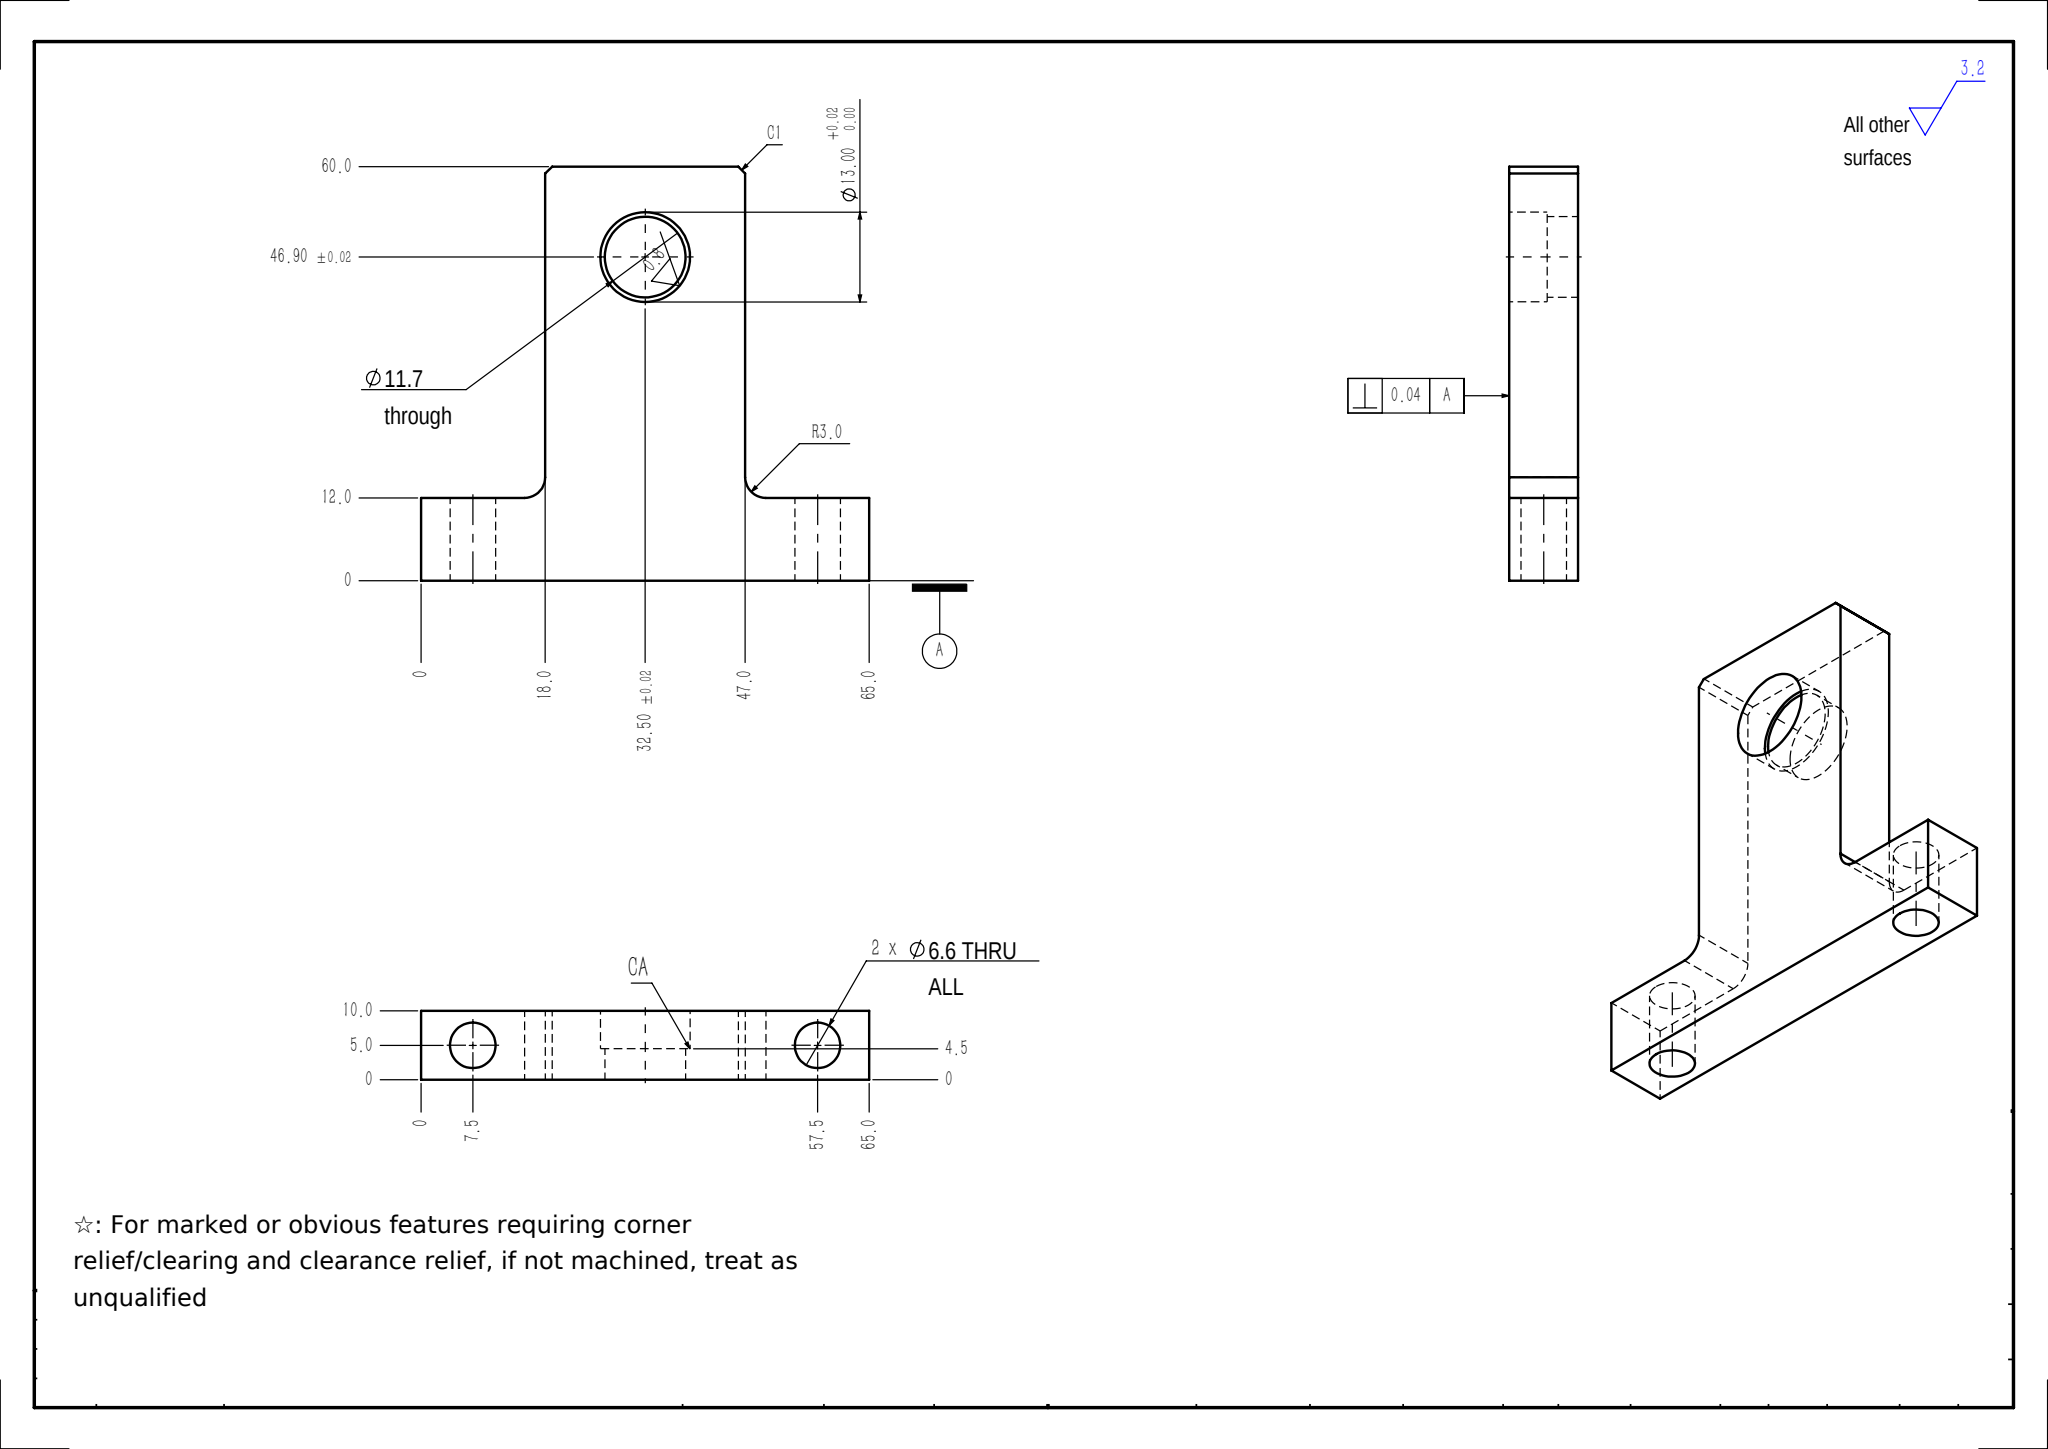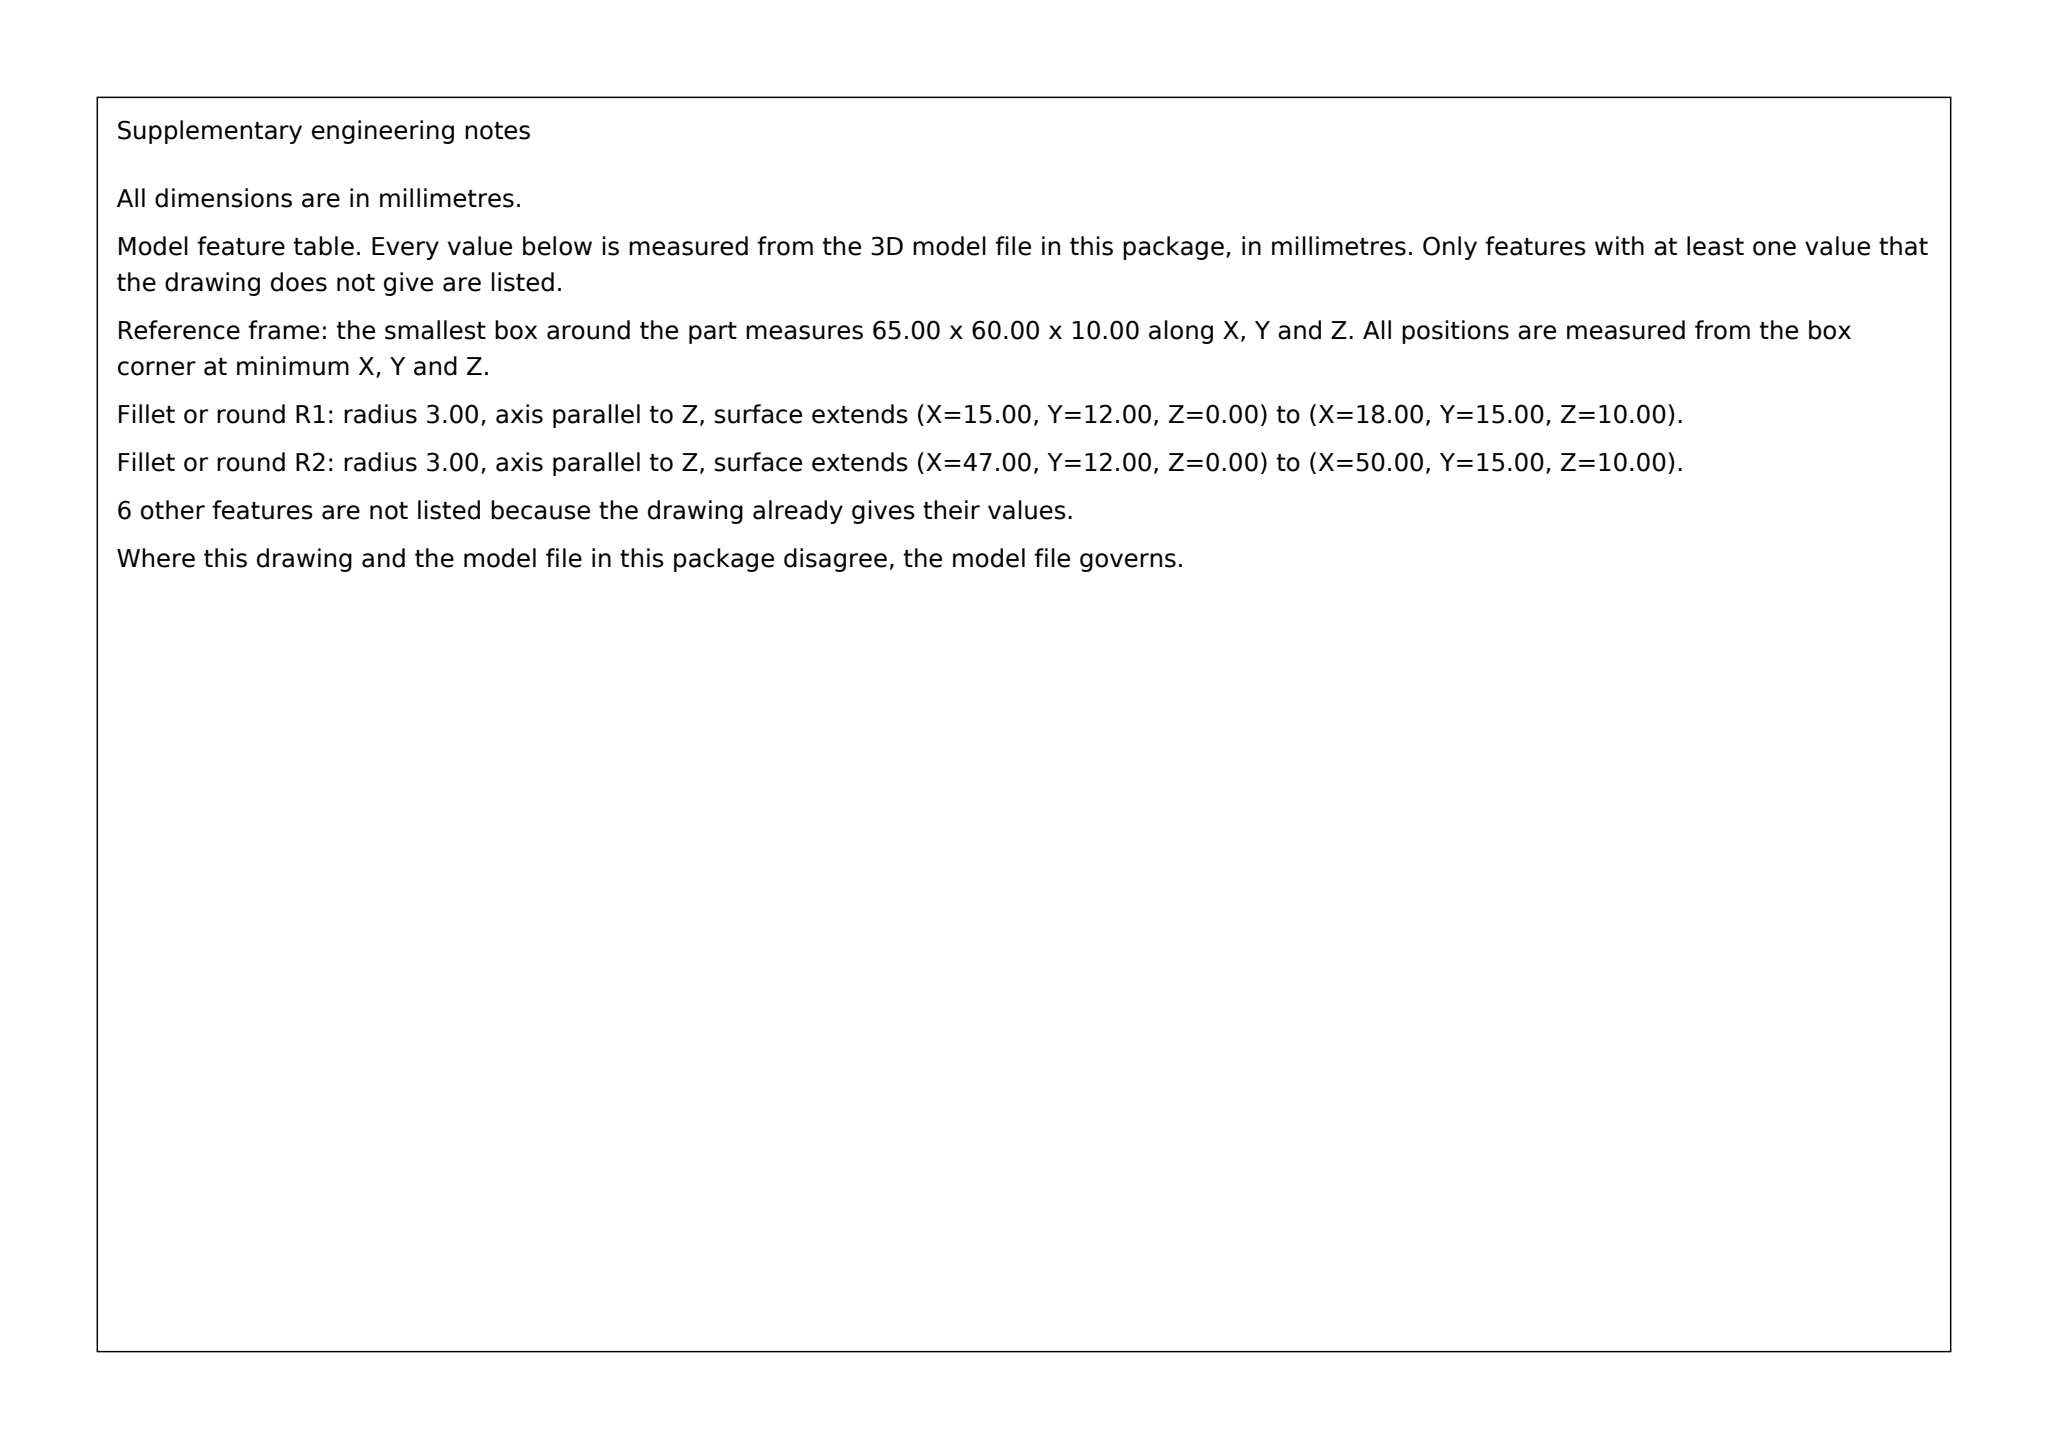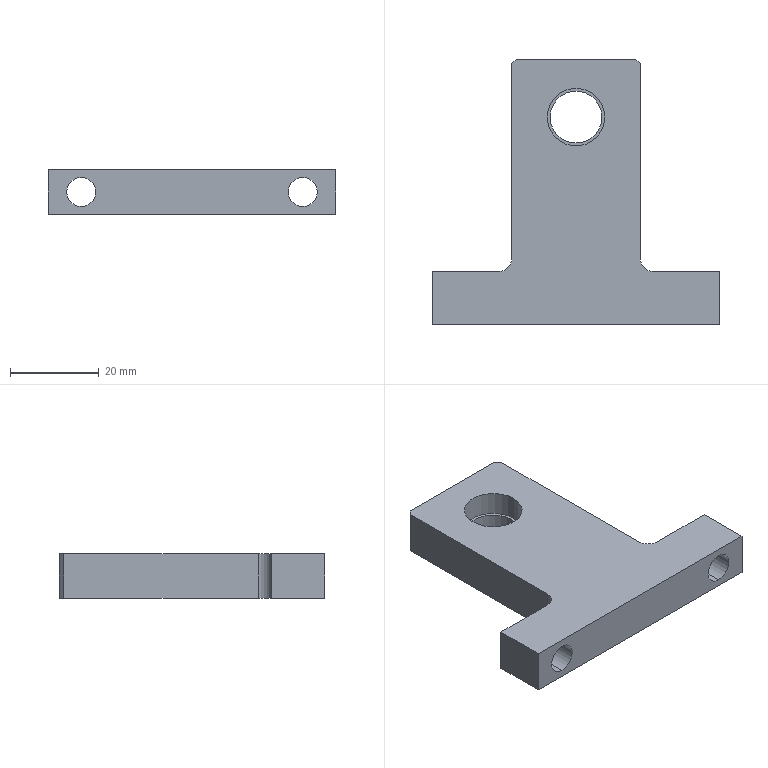Part | SolidWorks | mm | 1 solid | 23 faces | box 65 x 60 x 10 mm | volume 19714 mm3 | plane 13 | cylinder 10 | commonest cylinder face diameters 6.6 x4 11.7 x2 13 x2 6 x2
build123d program:
from build123d import *

# Parameters (mm, degrees)
BOSS_EXTRUDE1_DEPTH  = 5
FILLET1_R            = 3
SKETCH3_R            = 6.5
CUT_EXTRUDE1_DEPTH   = 46.346
SKETCH2_R            = 6.5
SKETCH2_R_2          = 5.85
BOSS_EXTRUDE2_DEPTH  = 4.5
M6_CLEARANCE_HOLE1_D = 6.6
CHAMFER1_SIZE        = 1


with BuildPart() as part:
    # Sketch1 → Boss-Extrude1 (new, symmetric)
    with BuildSketch(Plane.XY):
        Polygon((-14.5, 30), (-14.5, -18), (-32.5, -18), (-32.5, -30), (32.5, -30), (32.5, -18), (14.5, -18), (14.5, 30), align=None)
    extrude(amount=BOSS_EXTRUDE1_DEPTH, both=True)

    # Fillet1
    fillet1_edges = [part.edges().sort_by_distance(p)[0] for p in [
        (-14.5, -18, 0),
        (14.5, -18, 0),
    ]]
    fillet(fillet1_edges, radius=FILLET1_R)

    # Sketch3 → Cut-Extrude1 (cut, through all)
    with BuildSketch(Plane(origin=(0, 0, -5), x_dir=(-1, 0, 0), z_dir=(0, 0, -1))):
        with Locations((0, 16.9)):
            Circle(SKETCH3_R)
    extrude(amount=-CUT_EXTRUDE1_DEPTH, mode=Mode.SUBTRACT)

    # Sketch2 → Boss-Extrude2 (add)
    with BuildSketch(Plane(origin=(0, 0, -5), x_dir=(-1, 0, 0), z_dir=(0, 0, -1))):
        with Locations((0, 16.9)):
            Circle(SKETCH2_R)
        with Locations((0, 16.9)):
            Circle(SKETCH2_R_2, mode=Mode.SUBTRACT)
    extrude(amount=-BOSS_EXTRUDE2_DEPTH)

    # M6 Clearance Hole1 (through all)
    with Locations(Plane(origin=(0, -18, 0), x_dir=(1, 0, 0), z_dir=(0, 1, 0))):
        with Locations((-25, 0), (25, 0)):
            Hole(M6_CLEARANCE_HOLE1_D / 2)

    # Chamfer1
    chamfer1_edges = [part.edges().sort_by_distance(p)[0] for p in [
        (-14.5, 30, 0),
        (14.5, 30, 0),
    ]]
    chamfer(chamfer1_edges, length=CHAMFER1_SIZE)


solid = part.part
STEP:
#1=CARTESIAN_POINT('',(-25.,-30.,-3.3));
#2=VERTEX_POINT('',#1);
#3=CARTESIAN_POINT('',(-25.,-30.,3.3));
#4=VERTEX_POINT('',#3);
#5=CARTESIAN_POINT('',(-25.,-30.,0.));
#6=DIRECTION('',(0.,1.,0.));
#7=DIRECTION('',(0.,0.,1.));
#8=AXIS2_PLACEMENT_3D('',#5,#6,#7);
#9=CIRCLE('',#8,3.3);
#10=EDGE_CURVE('',#2,#4,#9,.T.);
#11=ORIENTED_EDGE('',*,*,#10,.F.);
#12=CARTESIAN_POINT('',(-25.,-18.,-3.3));
#13=VERTEX_POINT('',#12);
#14=CARTESIAN_POINT('',(-25.,-18.,-3.3));
#15=DIRECTION('',(0.,1.,0.));
#16=VECTOR('',#15,1000.);
#17=LINE('',#14,#16);
#18=EDGE_CURVE('',#2,#13,#17,.T.);
#19=ORIENTED_EDGE('',*,*,#18,.T.);
#20=CARTESIAN_POINT('',(-25.,-18.,3.3));
#21=VERTEX_POINT('',#20);
#22=CARTESIAN_POINT('',(-25.,-18.,0.));
#23=DIRECTION('',(0.,1.,0.));
#24=DIRECTION('',(0.,0.,1.));
#25=AXIS2_PLACEMENT_3D('',#22,#23,#24);
#26=CIRCLE('',#25,3.3);
#27=EDGE_CURVE('',#13,#21,#26,.T.);
#28=ORIENTED_EDGE('',*,*,#27,.T.);
#29=CARTESIAN_POINT('',(-25.,-18.,3.3));
#30=DIRECTION('',(0.,1.,0.));
#31=VECTOR('',#30,1000.);
#32=LINE('',#29,#31);
#33=EDGE_CURVE('',#4,#21,#32,.T.);
#34=ORIENTED_EDGE('',*,*,#33,.F.);
#35=EDGE_LOOP('',(#11,#19,#28,#34));
#36=FACE_OUTER_BOUND('',#35,.T.);
#37=CARTESIAN_POINT('',(-25.,-18.,0.));
#38=DIRECTION('',(0.,1.,0.));
#39=DIRECTION('',(0.,0.,1.));
#40=AXIS2_PLACEMENT_3D('',#37,#38,#39);
#41=CYLINDRICAL_SURFACE('',#40,3.3);
#42=ADVANCED_FACE('',(#36),#41,.F.);
#43=CARTESIAN_POINT('',(25.,-30.,-3.3));
#44=VERTEX_POINT('',#43);
#45=CARTESIAN_POINT('',(25.,-30.,3.3));
#46=VERTEX_POINT('',#45);
#47=CARTESIAN_POINT('',(25.,-30.,0.));
#48=DIRECTION('',(0.,1.,0.));
#49=DIRECTION('',(0.,0.,1.));
#50=AXIS2_PLACEMENT_3D('',#47,#48,#49);
#51=CIRCLE('',#50,3.3);
#52=EDGE_CURVE('',#44,#46,#51,.T.);
#53=ORIENTED_EDGE('',*,*,#52,.F.);
#54=CARTESIAN_POINT('',(25.,-18.,-3.3));
#55=VERTEX_POINT('',#54);
#56=CARTESIAN_POINT('',(25.,-18.,-3.3));
#57=DIRECTION('',(0.,1.,0.));
#58=VECTOR('',#57,1000.);
#59=LINE('',#56,#58);
#60=EDGE_CURVE('',#44,#55,#59,.T.);
#61=ORIENTED_EDGE('',*,*,#60,.T.);
#62=CARTESIAN_POINT('',(25.,-18.,3.3));
#63=VERTEX_POINT('',#62);
#64=CARTESIAN_POINT('',(25.,-18.,0.));
#65=DIRECTION('',(0.,1.,0.));
#66=DIRECTION('',(0.,0.,1.));
#67=AXIS2_PLACEMENT_3D('',#64,#65,#66);
#68=CIRCLE('',#67,3.3);
#69=EDGE_CURVE('',#55,#63,#68,.T.);
#70=ORIENTED_EDGE('',*,*,#69,.T.);
#71=CARTESIAN_POINT('',(25.,-18.,3.3));
#72=DIRECTION('',(0.,1.,0.));
#73=VECTOR('',#72,1000.);
#74=LINE('',#71,#73);
#75=EDGE_CURVE('',#46,#63,#74,.T.);
#76=ORIENTED_EDGE('',*,*,#75,.F.);
#77=EDGE_LOOP('',(#53,#61,#70,#76));
#78=FACE_OUTER_BOUND('',#77,.T.);
#79=CARTESIAN_POINT('',(25.,-18.,0.));
#80=DIRECTION('',(0.,1.,0.));
#81=DIRECTION('',(0.,0.,1.));
#82=AXIS2_PLACEMENT_3D('',#79,#80,#81);
#83=CYLINDRICAL_SURFACE('',#82,3.3);
#84=ADVANCED_FACE('',(#78),#83,.F.);
#85=CARTESIAN_POINT('',(5.85,16.9,-0.5));
#86=VERTEX_POINT('',#85);
#87=CARTESIAN_POINT('',(-5.85,16.9,-0.5));
#88=VERTEX_POINT('',#87);
#89=CARTESIAN_POINT('',(0.,16.9,-0.5));
#90=DIRECTION('',(0.,0.,-1.));
#91=DIRECTION('',(-1.,0.,0.));
#92=AXIS2_PLACEMENT_3D('',#89,#90,#91);
#93=CIRCLE('',#92,5.85);
#94=EDGE_CURVE('',#86,#88,#93,.T.);
#95=ORIENTED_EDGE('',*,*,#94,.F.);
#96=CARTESIAN_POINT('',(5.85,16.9,-5.));
#97=VERTEX_POINT('',#96);
#98=CARTESIAN_POINT('',(5.85,16.9,-0.5));
#99=DIRECTION('',(0.,0.,-1.));
#100=VECTOR('',#99,1000.);
#101=LINE('',#98,#100);
#102=EDGE_CURVE('',#86,#97,#101,.T.);
#103=ORIENTED_EDGE('',*,*,#102,.T.);
#104=CARTESIAN_POINT('',(-5.85,16.9,-5.));
#105=VERTEX_POINT('',#104);
#106=CARTESIAN_POINT('',(0.,16.9,-5.));
#107=DIRECTION('',(0.,0.,-1.));
#108=DIRECTION('',(-1.,0.,0.));
#109=AXIS2_PLACEMENT_3D('',#106,#107,#108);
#110=CIRCLE('',#109,5.85);
#111=EDGE_CURVE('',#97,#105,#110,.T.);
#112=ORIENTED_EDGE('',*,*,#111,.T.);
#113=CARTESIAN_POINT('',(-5.85,16.9,-0.5));
#114=DIRECTION('',(0.,0.,-1.));
#115=VECTOR('',#114,1000.);
#116=LINE('',#113,#115);
#117=EDGE_CURVE('',#88,#105,#116,.T.);
#118=ORIENTED_EDGE('',*,*,#117,.F.);
#119=EDGE_LOOP('',(#95,#103,#112,#118));
#120=FACE_OUTER_BOUND('',#119,.T.);
#121=CARTESIAN_POINT('',(0.,16.9,-0.5));
#122=DIRECTION('',(0.,0.,-1.));
#123=DIRECTION('',(-1.,0.,0.));
#124=AXIS2_PLACEMENT_3D('',#121,#122,#123);
#125=CYLINDRICAL_SURFACE('',#124,5.85);
#126=ADVANCED_FACE('',(#120),#125,.F.);
#127=CARTESIAN_POINT('',(6.5,16.9,5.));
#128=VERTEX_POINT('',#127);
#129=CARTESIAN_POINT('',(-6.5,16.9,5.));
#130=VERTEX_POINT('',#129);
#131=CARTESIAN_POINT('',(0.,16.9,5.));
#132=DIRECTION('',(0.,0.,-1.));
#133=DIRECTION('',(-1.,0.,0.));
#134=AXIS2_PLACEMENT_3D('',#131,#132,#133);
#135=CIRCLE('',#134,6.5);
#136=EDGE_CURVE('',#128,#130,#135,.T.);
#137=ORIENTED_EDGE('',*,*,#136,.F.);
#138=CARTESIAN_POINT('',(6.5,16.9,-0.5));
#139=VERTEX_POINT('',#138);
#140=CARTESIAN_POINT('',(6.5,16.9,5.));
#141=DIRECTION('',(0.,0.,-1.));
#142=VECTOR('',#141,1000.);
#143=LINE('',#140,#142);
#144=EDGE_CURVE('',#128,#139,#143,.T.);
#145=ORIENTED_EDGE('',*,*,#144,.T.);
#146=CARTESIAN_POINT('',(-6.5,16.9,-0.5));
#147=VERTEX_POINT('',#146);
#148=CARTESIAN_POINT('',(0.,16.9,-0.5));
#149=DIRECTION('',(0.,0.,1.));
#150=DIRECTION('',(-1.,0.,0.));
#151=AXIS2_PLACEMENT_3D('',#148,#149,#150);
#152=CIRCLE('',#151,6.5);
#153=EDGE_CURVE('',#147,#139,#152,.T.);
#154=ORIENTED_EDGE('',*,*,#153,.F.);
#155=CARTESIAN_POINT('',(-6.5,16.9,5.));
#156=DIRECTION('',(0.,0.,-1.));
#157=VECTOR('',#156,1000.);
#158=LINE('',#155,#157);
#159=EDGE_CURVE('',#130,#147,#158,.T.);
#160=ORIENTED_EDGE('',*,*,#159,.F.);
#161=EDGE_LOOP('',(#137,#145,#154,#160));
#162=FACE_OUTER_BOUND('',#161,.T.);
#163=CARTESIAN_POINT('',(0.,16.9,5.));
#164=DIRECTION('',(0.,0.,-1.));
#165=DIRECTION('',(-1.,0.,0.));
#166=AXIS2_PLACEMENT_3D('',#163,#164,#165);
#167=CYLINDRICAL_SURFACE('',#166,6.5);
#168=ADVANCED_FACE('',(#162),#167,.F.);
#169=ORIENTED_EDGE('',*,*,#144,.F.);
#170=CARTESIAN_POINT('',(0.,16.9,5.));
#171=DIRECTION('',(0.,0.,-1.));
#172=DIRECTION('',(-1.,0.,0.));
#173=AXIS2_PLACEMENT_3D('',#170,#171,#172);
#174=CIRCLE('',#173,6.5);
#175=EDGE_CURVE('',#130,#128,#174,.T.);
#176=ORIENTED_EDGE('',*,*,#175,.F.);
#177=ORIENTED_EDGE('',*,*,#159,.T.);
#178=CARTESIAN_POINT('',(0.,16.9,-0.5));
#179=DIRECTION('',(0.,0.,1.));
#180=DIRECTION('',(-1.,0.,0.));
#181=AXIS2_PLACEMENT_3D('',#178,#179,#180);
#182=CIRCLE('',#181,6.5);
#183=EDGE_CURVE('',#139,#147,#182,.T.);
#184=ORIENTED_EDGE('',*,*,#183,.F.);
#185=EDGE_LOOP('',(#169,#176,#177,#184));
#186=FACE_OUTER_BOUND('',#185,.T.);
#187=CARTESIAN_POINT('',(0.,16.9,5.));
#188=DIRECTION('',(0.,0.,-1.));
#189=DIRECTION('',(-1.,0.,0.));
#190=AXIS2_PLACEMENT_3D('',#187,#188,#189);
#191=CYLINDRICAL_SURFACE('',#190,6.5);
#192=ADVANCED_FACE('',(#186),#191,.F.);
#193=CARTESIAN_POINT('',(-32.5,-18.,-5.));
#194=VERTEX_POINT('',#193);
#195=CARTESIAN_POINT('',(-32.5,-30.,-5.));
#196=VERTEX_POINT('',#195);
#197=CARTESIAN_POINT('',(-32.5,-30.,-5.));
#198=DIRECTION('',(-0.,-1.,0.));
#199=VECTOR('',#198,1000.);
#200=LINE('',#197,#199);
#201=EDGE_CURVE('',#194,#196,#200,.T.);
#202=ORIENTED_EDGE('',*,*,#201,.T.);
#203=CARTESIAN_POINT('',(-32.5,-30.,5.));
#204=VERTEX_POINT('',#203);
#205=CARTESIAN_POINT('',(-32.5,-30.,5.));
#206=DIRECTION('',(0.,0.,-1.));
#207=VECTOR('',#206,1000.);
#208=LINE('',#205,#207);
#209=EDGE_CURVE('',#204,#196,#208,.T.);
#210=ORIENTED_EDGE('',*,*,#209,.F.);
#211=CARTESIAN_POINT('',(-32.5,-18.,5.));
#212=VERTEX_POINT('',#211);
#213=CARTESIAN_POINT('',(-32.5,-30.,5.));
#214=DIRECTION('',(-0.,-1.,0.));
#215=VECTOR('',#214,1000.);
#216=LINE('',#213,#215);
#217=EDGE_CURVE('',#212,#204,#216,.T.);
#218=ORIENTED_EDGE('',*,*,#217,.F.);
#219=CARTESIAN_POINT('',(-32.5,-18.,5.));
#220=DIRECTION('',(0.,0.,-1.));
#221=VECTOR('',#220,1000.);
#222=LINE('',#219,#221);
#223=EDGE_CURVE('',#212,#194,#222,.T.);
#224=ORIENTED_EDGE('',*,*,#223,.T.);
#225=EDGE_LOOP('',(#202,#210,#218,#224));
#226=FACE_OUTER_BOUND('',#225,.T.);
#227=CARTESIAN_POINT('',(-32.5,-30.,5.));
#228=DIRECTION('',(1.,-0.,0.));
#229=DIRECTION('',(0.,1.,0.));
#230=AXIS2_PLACEMENT_3D('',#227,#228,#229);
#231=PLANE('',#230);
#232=ADVANCED_FACE('',(#226),#231,.F.);
#233=CARTESIAN_POINT('',(-25.,-30.,0.));
#234=DIRECTION('',(0.,1.,0.));
#235=DIRECTION('',(0.,0.,1.));
#236=AXIS2_PLACEMENT_3D('',#233,#234,#235);
#237=CIRCLE('',#236,3.3);
#238=EDGE_CURVE('',#4,#2,#237,.T.);
#239=ORIENTED_EDGE('',*,*,#238,.T.);
#240=ORIENTED_EDGE('',*,*,#10,.T.);
#241=EDGE_LOOP('',(#239,#240));
#242=FACE_BOUND('',#241,.T.);
#243=CARTESIAN_POINT('',(25.,-30.,0.));
#244=DIRECTION('',(0.,1.,0.));
#245=DIRECTION('',(0.,0.,1.));
#246=AXIS2_PLACEMENT_3D('',#243,#244,#245);
#247=CIRCLE('',#246,3.3);
#248=EDGE_CURVE('',#46,#44,#247,.T.);
#249=ORIENTED_EDGE('',*,*,#248,.T.);
#250=ORIENTED_EDGE('',*,*,#52,.T.);
#251=EDGE_LOOP('',(#249,#250));
#252=FACE_BOUND('',#251,.T.);
#253=CARTESIAN_POINT('',(32.5,-30.,-5.));
#254=VERTEX_POINT('',#253);
#255=CARTESIAN_POINT('',(-32.5,-30.,-5.));
#256=DIRECTION('',(1.,0.,0.));
#257=VECTOR('',#256,1000.);
#258=LINE('',#255,#257);
#259=EDGE_CURVE('',#196,#254,#258,.T.);
#260=ORIENTED_EDGE('',*,*,#259,.T.);
#261=CARTESIAN_POINT('',(32.5,-30.,5.));
#262=VERTEX_POINT('',#261);
#263=CARTESIAN_POINT('',(32.5,-30.,5.));
#264=DIRECTION('',(0.,0.,-1.));
#265=VECTOR('',#264,1000.);
#266=LINE('',#263,#265);
#267=EDGE_CURVE('',#262,#254,#266,.T.);
#268=ORIENTED_EDGE('',*,*,#267,.F.);
#269=CARTESIAN_POINT('',(-32.5,-30.,5.));
#270=DIRECTION('',(1.,0.,0.));
#271=VECTOR('',#270,1000.);
#272=LINE('',#269,#271);
#273=EDGE_CURVE('',#204,#262,#272,.T.);
#274=ORIENTED_EDGE('',*,*,#273,.F.);
#275=ORIENTED_EDGE('',*,*,#209,.T.);
#276=EDGE_LOOP('',(#260,#268,#274,#275));
#277=FACE_OUTER_BOUND('',#276,.T.);
#278=CARTESIAN_POINT('',(-32.5,-30.,5.));
#279=DIRECTION('',(-0.,1.,0.));
#280=DIRECTION('',(-1.,-0.,0.));
#281=AXIS2_PLACEMENT_3D('',#278,#279,#280);
#282=PLANE('',#281);
#283=ADVANCED_FACE('',(#242,#252,#277),#282,.F.);
#284=CARTESIAN_POINT('',(32.5,-18.,-5.));
#285=VERTEX_POINT('',#284);
#286=CARTESIAN_POINT('',(32.5,-30.,-5.));
#287=DIRECTION('',(-0.,1.,0.));
#288=VECTOR('',#287,1000.);
#289=LINE('',#286,#288);
#290=EDGE_CURVE('',#254,#285,#289,.T.);
#291=ORIENTED_EDGE('',*,*,#290,.T.);
#292=CARTESIAN_POINT('',(32.5,-18.,5.));
#293=VERTEX_POINT('',#292);
#294=CARTESIAN_POINT('',(32.5,-18.,5.));
#295=DIRECTION('',(0.,0.,-1.));
#296=VECTOR('',#295,1000.);
#297=LINE('',#294,#296);
#298=EDGE_CURVE('',#293,#285,#297,.T.);
#299=ORIENTED_EDGE('',*,*,#298,.F.);
#300=CARTESIAN_POINT('',(32.5,-30.,5.));
#301=DIRECTION('',(-0.,1.,0.));
#302=VECTOR('',#301,1000.);
#303=LINE('',#300,#302);
#304=EDGE_CURVE('',#262,#293,#303,.T.);
#305=ORIENTED_EDGE('',*,*,#304,.F.);
#306=ORIENTED_EDGE('',*,*,#267,.T.);
#307=EDGE_LOOP('',(#291,#299,#305,#306));
#308=FACE_OUTER_BOUND('',#307,.T.);
#309=CARTESIAN_POINT('',(32.5,-30.,5.));
#310=DIRECTION('',(-1.,-0.,0.));
#311=DIRECTION('',(0.,-1.,0.));
#312=AXIS2_PLACEMENT_3D('',#309,#310,#311);
#313=PLANE('',#312);
#314=ADVANCED_FACE('',(#308),#313,.F.);
#315=CARTESIAN_POINT('',(25.,-18.,0.));
#316=DIRECTION('',(0.,1.,0.));
#317=DIRECTION('',(0.,0.,1.));
#318=AXIS2_PLACEMENT_3D('',#315,#316,#317);
#319=CIRCLE('',#318,3.3);
#320=EDGE_CURVE('',#63,#55,#319,.T.);
#321=ORIENTED_EDGE('',*,*,#320,.F.);
#322=ORIENTED_EDGE('',*,*,#69,.F.);
#323=EDGE_LOOP('',(#321,#322));
#324=FACE_BOUND('',#323,.T.);
#325=CARTESIAN_POINT('',(17.5,-18.,-5.));
#326=VERTEX_POINT('',#325);
#327=CARTESIAN_POINT('',(14.5,-18.,-5.));
#328=DIRECTION('',(-1.,0.,0.));
#329=VECTOR('',#328,1000.);
#330=LINE('',#327,#329);
#331=EDGE_CURVE('',#285,#326,#330,.T.);
#332=ORIENTED_EDGE('',*,*,#331,.T.);
#333=CARTESIAN_POINT('',(17.5,-18.,5.));
#334=VERTEX_POINT('',#333);
#335=CARTESIAN_POINT('',(17.5,-18.,5.));
#336=DIRECTION('',(0.,0.,1.));
#337=VECTOR('',#336,1000.);
#338=LINE('',#335,#337);
#339=EDGE_CURVE('',#326,#334,#338,.T.);
#340=ORIENTED_EDGE('',*,*,#339,.T.);
#341=CARTESIAN_POINT('',(14.5,-18.,5.));
#342=DIRECTION('',(-1.,0.,0.));
#343=VECTOR('',#342,1000.);
#344=LINE('',#341,#343);
#345=EDGE_CURVE('',#293,#334,#344,.T.);
#346=ORIENTED_EDGE('',*,*,#345,.F.);
#347=ORIENTED_EDGE('',*,*,#298,.T.);
#348=EDGE_LOOP('',(#332,#340,#346,#347));
#349=FACE_OUTER_BOUND('',#348,.T.);
#350=CARTESIAN_POINT('',(14.5,-18.,5.));
#351=DIRECTION('',(0.,-1.,0.));
#352=DIRECTION('',(0.,0.,-1.));
#353=AXIS2_PLACEMENT_3D('',#350,#351,#352);
#354=PLANE('',#353);
#355=ADVANCED_FACE('',(#324,#349),#354,.F.);
#356=CARTESIAN_POINT('',(14.5,-15.,-5.));
#357=VERTEX_POINT('',#356);
#358=CARTESIAN_POINT('',(14.5,29.,-5.));
#359=VERTEX_POINT('',#358);
#360=CARTESIAN_POINT('',(14.5,30.,-5.));
#361=DIRECTION('',(-0.,1.,0.));
#362=VECTOR('',#361,1000.);
#363=LINE('',#360,#362);
#364=EDGE_CURVE('',#357,#359,#363,.T.);
#365=ORIENTED_EDGE('',*,*,#364,.T.);
#366=CARTESIAN_POINT('',(14.5,29.,5.));
#367=VERTEX_POINT('',#366);
#368=CARTESIAN_POINT('',(14.5,29.,5.));
#369=DIRECTION('',(0.,0.,1.));
#370=VECTOR('',#369,1000.);
#371=LINE('',#368,#370);
#372=EDGE_CURVE('',#359,#367,#371,.T.);
#373=ORIENTED_EDGE('',*,*,#372,.T.);
#374=CARTESIAN_POINT('',(14.5,-15.,5.));
#375=VERTEX_POINT('',#374);
#376=CARTESIAN_POINT('',(14.5,30.,5.));
#377=DIRECTION('',(-0.,1.,0.));
#378=VECTOR('',#377,1000.);
#379=LINE('',#376,#378);
#380=EDGE_CURVE('',#375,#367,#379,.T.);
#381=ORIENTED_EDGE('',*,*,#380,.F.);
#382=CARTESIAN_POINT('',(14.5,-15.,-5.));
#383=DIRECTION('',(0.,0.,-1.));
#384=VECTOR('',#383,1000.);
#385=LINE('',#382,#384);
#386=EDGE_CURVE('',#375,#357,#385,.T.);
#387=ORIENTED_EDGE('',*,*,#386,.T.);
#388=EDGE_LOOP('',(#365,#373,#381,#387));
#389=FACE_OUTER_BOUND('',#388,.T.);
#390=CARTESIAN_POINT('',(14.5,30.,5.));
#391=DIRECTION('',(-1.,-0.,0.));
#392=DIRECTION('',(0.,-1.,0.));
#393=AXIS2_PLACEMENT_3D('',#390,#391,#392);
#394=PLANE('',#393);
#395=ADVANCED_FACE('',(#389),#394,.F.);
#396=CARTESIAN_POINT('',(13.5,30.,5.));
#397=VERTEX_POINT('',#396);
#398=CARTESIAN_POINT('',(-13.5,30.,5.));
#399=VERTEX_POINT('',#398);
#400=CARTESIAN_POINT('',(-14.5,30.,5.));
#401=DIRECTION('',(-1.,-0.,0.));
#402=VECTOR('',#401,1000.);
#403=LINE('',#400,#402);
#404=EDGE_CURVE('',#397,#399,#403,.T.);
#405=ORIENTED_EDGE('',*,*,#404,.F.);
#406=CARTESIAN_POINT('',(13.5,30.,-5.));
#407=VERTEX_POINT('',#406);
#408=CARTESIAN_POINT('',(13.5,30.,5.));
#409=DIRECTION('',(0.,0.,-1.));
#410=VECTOR('',#409,1000.);
#411=LINE('',#408,#410);
#412=EDGE_CURVE('',#397,#407,#411,.T.);
#413=ORIENTED_EDGE('',*,*,#412,.T.);
#414=CARTESIAN_POINT('',(-13.5,30.,-5.));
#415=VERTEX_POINT('',#414);
#416=CARTESIAN_POINT('',(-14.5,30.,-5.));
#417=DIRECTION('',(-1.,-0.,0.));
#418=VECTOR('',#417,1000.);
#419=LINE('',#416,#418);
#420=EDGE_CURVE('',#407,#415,#419,.T.);
#421=ORIENTED_EDGE('',*,*,#420,.T.);
#422=CARTESIAN_POINT('',(-13.5,30.,5.));
#423=DIRECTION('',(0.,0.,1.));
#424=VECTOR('',#423,1000.);
#425=LINE('',#422,#424);
#426=EDGE_CURVE('',#415,#399,#425,.T.);
#427=ORIENTED_EDGE('',*,*,#426,.T.);
#428=EDGE_LOOP('',(#405,#413,#421,#427));
#429=FACE_OUTER_BOUND('',#428,.T.);
#430=CARTESIAN_POINT('',(-14.5,30.,5.));
#431=DIRECTION('',(0.,-1.,0.));
#432=DIRECTION('',(1.,0.,0.));
#433=AXIS2_PLACEMENT_3D('',#430,#431,#432);
#434=PLANE('',#433);
#435=ADVANCED_FACE('',(#429),#434,.F.);
#436=CARTESIAN_POINT('',(-14.5,29.,5.));
#437=VERTEX_POINT('',#436);
#438=CARTESIAN_POINT('',(-14.5,-15.,5.));
#439=VERTEX_POINT('',#438);
#440=CARTESIAN_POINT('',(-14.5,30.,5.));
#441=DIRECTION('',(0.,-1.,0.));
#442=VECTOR('',#441,1000.);
#443=LINE('',#440,#442);
#444=EDGE_CURVE('',#437,#439,#443,.T.);
#445=ORIENTED_EDGE('',*,*,#444,.F.);
#446=CARTESIAN_POINT('',(-14.5,29.,-5.));
#447=VERTEX_POINT('',#446);
#448=CARTESIAN_POINT('',(-14.5,29.,5.));
#449=DIRECTION('',(0.,0.,-1.));
#450=VECTOR('',#449,1000.);
#451=LINE('',#448,#450);
#452=EDGE_CURVE('',#437,#447,#451,.T.);
#453=ORIENTED_EDGE('',*,*,#452,.T.);
#454=CARTESIAN_POINT('',(-14.5,-15.,-5.));
#455=VERTEX_POINT('',#454);
#456=CARTESIAN_POINT('',(-14.5,30.,-5.));
#457=DIRECTION('',(0.,-1.,0.));
#458=VECTOR('',#457,1000.);
#459=LINE('',#456,#458);
#460=EDGE_CURVE('',#447,#455,#459,.T.);
#461=ORIENTED_EDGE('',*,*,#460,.T.);
#462=CARTESIAN_POINT('',(-14.5,-15.,5.));
#463=DIRECTION('',(0.,0.,1.));
#464=VECTOR('',#463,1000.);
#465=LINE('',#462,#464);
#466=EDGE_CURVE('',#455,#439,#465,.T.);
#467=ORIENTED_EDGE('',*,*,#466,.T.);
#468=EDGE_LOOP('',(#445,#453,#461,#467));
#469=FACE_OUTER_BOUND('',#468,.T.);
#470=CARTESIAN_POINT('',(-14.5,30.,5.));
#471=DIRECTION('',(1.,0.,0.));
#472=DIRECTION('',(-0.,1.,0.));
#473=AXIS2_PLACEMENT_3D('',#470,#471,#472);
#474=PLANE('',#473);
#475=ADVANCED_FACE('',(#469),#474,.F.);
#476=CARTESIAN_POINT('',(-25.,-18.,0.));
#477=DIRECTION('',(0.,1.,0.));
#478=DIRECTION('',(0.,0.,1.));
#479=AXIS2_PLACEMENT_3D('',#476,#477,#478);
#480=CIRCLE('',#479,3.3);
#481=EDGE_CURVE('',#21,#13,#480,.T.);
#482=ORIENTED_EDGE('',*,*,#481,.F.);
#483=ORIENTED_EDGE('',*,*,#27,.F.);
#484=EDGE_LOOP('',(#482,#483));
#485=FACE_BOUND('',#484,.T.);
#486=CARTESIAN_POINT('',(-17.5,-18.,5.));
#487=VERTEX_POINT('',#486);
#488=CARTESIAN_POINT('',(-14.5,-18.,5.));
#489=DIRECTION('',(-1.,-0.,0.));
#490=VECTOR('',#489,1000.);
#491=LINE('',#488,#490);
#492=EDGE_CURVE('',#487,#212,#491,.T.);
#493=ORIENTED_EDGE('',*,*,#492,.F.);
#494=CARTESIAN_POINT('',(-17.5,-18.,-5.));
#495=VERTEX_POINT('',#494);
#496=CARTESIAN_POINT('',(-17.5,-18.,-5.));
#497=DIRECTION('',(0.,0.,-1.));
#498=VECTOR('',#497,1000.);
#499=LINE('',#496,#498);
#500=EDGE_CURVE('',#487,#495,#499,.T.);
#501=ORIENTED_EDGE('',*,*,#500,.T.);
#502=CARTESIAN_POINT('',(-14.5,-18.,-5.));
#503=DIRECTION('',(-1.,-0.,0.));
#504=VECTOR('',#503,1000.);
#505=LINE('',#502,#504);
#506=EDGE_CURVE('',#495,#194,#505,.T.);
#507=ORIENTED_EDGE('',*,*,#506,.T.);
#508=ORIENTED_EDGE('',*,*,#223,.F.);
#509=EDGE_LOOP('',(#493,#501,#507,#508));
#510=FACE_OUTER_BOUND('',#509,.T.);
#511=CARTESIAN_POINT('',(-14.5,-18.,5.));
#512=DIRECTION('',(0.,-1.,0.));
#513=DIRECTION('',(1.,0.,0.));
#514=AXIS2_PLACEMENT_3D('',#511,#512,#513);
#515=PLANE('',#514);
#516=ADVANCED_FACE('',(#485,#510),#515,.F.);
#517=ORIENTED_EDGE('',*,*,#175,.T.);
#518=ORIENTED_EDGE('',*,*,#136,.T.);
#519=EDGE_LOOP('',(#517,#518));
#520=FACE_BOUND('',#519,.T.);
#521=ORIENTED_EDGE('',*,*,#380,.T.);
#522=CARTESIAN_POINT('',(21.75,21.75,5.));
#523=DIRECTION('',(-0.7071,0.7071,0.));
#524=VECTOR('',#523,1000.);
#525=LINE('',#522,#524);
#526=EDGE_CURVE('',#367,#397,#525,.T.);
#527=ORIENTED_EDGE('',*,*,#526,.T.);
#528=ORIENTED_EDGE('',*,*,#404,.T.);
#529=CARTESIAN_POINT('',(-21.75,21.75,5.));
#530=DIRECTION('',(-0.7071,-0.7071,0.));
#531=VECTOR('',#530,1000.);
#532=LINE('',#529,#531);
#533=EDGE_CURVE('',#399,#437,#532,.T.);
#534=ORIENTED_EDGE('',*,*,#533,.T.);
#535=ORIENTED_EDGE('',*,*,#444,.T.);
#536=CARTESIAN_POINT('',(-17.5,-15.,5.));
#537=DIRECTION('',(0.,0.,-1.));
#538=DIRECTION('',(1.,0.,0.));
#539=AXIS2_PLACEMENT_3D('',#536,#537,#538);
#540=CIRCLE('',#539,3.);
#541=EDGE_CURVE('',#439,#487,#540,.T.);
#542=ORIENTED_EDGE('',*,*,#541,.T.);
#543=ORIENTED_EDGE('',*,*,#492,.T.);
#544=ORIENTED_EDGE('',*,*,#217,.T.);
#545=ORIENTED_EDGE('',*,*,#273,.T.);
#546=ORIENTED_EDGE('',*,*,#304,.T.);
#547=ORIENTED_EDGE('',*,*,#345,.T.);
#548=CARTESIAN_POINT('',(17.5,-15.,5.));
#549=DIRECTION('',(0.,0.,-1.));
#550=DIRECTION('',(1.,0.,0.));
#551=AXIS2_PLACEMENT_3D('',#548,#549,#550);
#552=CIRCLE('',#551,3.);
#553=EDGE_CURVE('',#334,#375,#552,.T.);
#554=ORIENTED_EDGE('',*,*,#553,.T.);
#555=EDGE_LOOP('',(#521,#527,#528,#534,#535,#542,#543,#544,#545,#546,#547,#554));
#556=FACE_OUTER_BOUND('',#555,.T.);
#557=CARTESIAN_POINT('',(0.,0.,5.));
#558=DIRECTION('',(0.,0.,1.));
#559=DIRECTION('',(1.,0.,0.));
#560=AXIS2_PLACEMENT_3D('',#557,#558,#559);
#561=PLANE('',#560);
#562=ADVANCED_FACE('',(#520,#556),#561,.T.);
#563=ORIENTED_EDGE('',*,*,#420,.F.);
#564=CARTESIAN_POINT('',(13.5,30.,-5.));
#565=DIRECTION('',(0.7071,-0.7071,0.));
#566=VECTOR('',#565,1000.);
#567=LINE('',#564,#566);
#568=EDGE_CURVE('',#407,#359,#567,.T.);
#569=ORIENTED_EDGE('',*,*,#568,.T.);
#570=ORIENTED_EDGE('',*,*,#364,.F.);
#571=CARTESIAN_POINT('',(17.5,-15.,-5.));
#572=DIRECTION('',(0.,0.,1.));
#573=DIRECTION('',(1.,0.,0.));
#574=AXIS2_PLACEMENT_3D('',#571,#572,#573);
#575=CIRCLE('',#574,3.);
#576=EDGE_CURVE('',#357,#326,#575,.T.);
#577=ORIENTED_EDGE('',*,*,#576,.T.);
#578=ORIENTED_EDGE('',*,*,#331,.F.);
#579=ORIENTED_EDGE('',*,*,#290,.F.);
#580=ORIENTED_EDGE('',*,*,#259,.F.);
#581=ORIENTED_EDGE('',*,*,#201,.F.);
#582=ORIENTED_EDGE('',*,*,#506,.F.);
#583=CARTESIAN_POINT('',(-17.5,-15.,-5.));
#584=DIRECTION('',(0.,0.,1.));
#585=DIRECTION('',(1.,0.,0.));
#586=AXIS2_PLACEMENT_3D('',#583,#584,#585);
#587=CIRCLE('',#586,3.);
#588=EDGE_CURVE('',#495,#455,#587,.T.);
#589=ORIENTED_EDGE('',*,*,#588,.T.);
#590=ORIENTED_EDGE('',*,*,#460,.F.);
#591=CARTESIAN_POINT('',(-14.5,29.,-5.));
#592=DIRECTION('',(0.7071,0.7071,0.));
#593=VECTOR('',#592,1000.);
#594=LINE('',#591,#593);
#595=EDGE_CURVE('',#447,#415,#594,.T.);
#596=ORIENTED_EDGE('',*,*,#595,.T.);
#597=EDGE_LOOP('',(#563,#569,#570,#577,#578,#579,#580,#581,#582,#589,#590,#596));
#598=FACE_OUTER_BOUND('',#597,.T.);
#599=CARTESIAN_POINT('',(0.,16.9,-5.));
#600=DIRECTION('',(0.,0.,-1.));
#601=DIRECTION('',(-1.,0.,0.));
#602=AXIS2_PLACEMENT_3D('',#599,#600,#601);
#603=CIRCLE('',#602,5.85);
#604=EDGE_CURVE('',#105,#97,#603,.T.);
#605=ORIENTED_EDGE('',*,*,#604,.F.);
#606=ORIENTED_EDGE('',*,*,#111,.F.);
#607=EDGE_LOOP('',(#605,#606));
#608=FACE_BOUND('',#607,.T.);
#609=CARTESIAN_POINT('',(0.,0.,-5.));
#610=DIRECTION('',(0.,0.,1.));
#611=DIRECTION('',(1.,0.,0.));
#612=AXIS2_PLACEMENT_3D('',#609,#610,#611);
#613=PLANE('',#612);
#614=ADVANCED_FACE('',(#598,#608),#613,.F.);
#615=ORIENTED_EDGE('',*,*,#553,.F.);
#616=ORIENTED_EDGE('',*,*,#339,.F.);
#617=ORIENTED_EDGE('',*,*,#576,.F.);
#618=ORIENTED_EDGE('',*,*,#386,.F.);
#619=EDGE_LOOP('',(#615,#616,#617,#618));
#620=FACE_OUTER_BOUND('',#619,.T.);
#621=CARTESIAN_POINT('',(17.5,-15.,5.));
#622=DIRECTION('',(0.,0.,1.));
#623=DIRECTION('',(1.,0.,0.));
#624=AXIS2_PLACEMENT_3D('',#621,#622,#623);
#625=CYLINDRICAL_SURFACE('',#624,3.);
#626=ADVANCED_FACE('',(#620),#625,.F.);
#627=ORIENTED_EDGE('',*,*,#541,.F.);
#628=ORIENTED_EDGE('',*,*,#466,.F.);
#629=ORIENTED_EDGE('',*,*,#588,.F.);
#630=ORIENTED_EDGE('',*,*,#500,.F.);
#631=EDGE_LOOP('',(#627,#628,#629,#630));
#632=FACE_OUTER_BOUND('',#631,.T.);
#633=CARTESIAN_POINT('',(-17.5,-15.,5.));
#634=DIRECTION('',(0.,0.,1.));
#635=DIRECTION('',(1.,0.,0.));
#636=AXIS2_PLACEMENT_3D('',#633,#634,#635);
#637=CYLINDRICAL_SURFACE('',#636,3.);
#638=ADVANCED_FACE('',(#632),#637,.F.);
#639=CARTESIAN_POINT('',(0.,16.9,-0.5));
#640=DIRECTION('',(0.,0.,-1.));
#641=DIRECTION('',(-1.,0.,0.));
#642=AXIS2_PLACEMENT_3D('',#639,#640,#641);
#643=CIRCLE('',#642,5.85);
#644=EDGE_CURVE('',#88,#86,#643,.T.);
#645=ORIENTED_EDGE('',*,*,#644,.T.);
#646=ORIENTED_EDGE('',*,*,#94,.T.);
#647=EDGE_LOOP('',(#645,#646));
#648=FACE_BOUND('',#647,.T.);
#649=ORIENTED_EDGE('',*,*,#153,.T.);
#650=ORIENTED_EDGE('',*,*,#183,.T.);
#651=EDGE_LOOP('',(#649,#650));
#652=FACE_OUTER_BOUND('',#651,.T.);
#653=CARTESIAN_POINT('',(0.,16.9,-0.5));
#654=DIRECTION('',(0.,0.,-1.));
#655=DIRECTION('',(-1.,0.,0.));
#656=AXIS2_PLACEMENT_3D('',#653,#654,#655);
#657=PLANE('',#656);
#658=ADVANCED_FACE('',(#648,#652),#657,.F.);
#659=ORIENTED_EDGE('',*,*,#102,.F.);
#660=ORIENTED_EDGE('',*,*,#644,.F.);
#661=ORIENTED_EDGE('',*,*,#117,.T.);
#662=ORIENTED_EDGE('',*,*,#604,.T.);
#663=EDGE_LOOP('',(#659,#660,#661,#662));
#664=FACE_OUTER_BOUND('',#663,.T.);
#665=CARTESIAN_POINT('',(0.,16.9,-0.5));
#666=DIRECTION('',(0.,0.,-1.));
#667=DIRECTION('',(-1.,0.,0.));
#668=AXIS2_PLACEMENT_3D('',#665,#666,#667);
#669=CYLINDRICAL_SURFACE('',#668,5.85);
#670=ADVANCED_FACE('',(#664),#669,.F.);
#671=ORIENTED_EDGE('',*,*,#60,.F.);
#672=ORIENTED_EDGE('',*,*,#248,.F.);
#673=ORIENTED_EDGE('',*,*,#75,.T.);
#674=ORIENTED_EDGE('',*,*,#320,.T.);
#675=EDGE_LOOP('',(#671,#672,#673,#674));
#676=FACE_OUTER_BOUND('',#675,.T.);
#677=CARTESIAN_POINT('',(25.,-18.,0.));
#678=DIRECTION('',(0.,1.,0.));
#679=DIRECTION('',(0.,0.,1.));
#680=AXIS2_PLACEMENT_3D('',#677,#678,#679);
#681=CYLINDRICAL_SURFACE('',#680,3.3);
#682=ADVANCED_FACE('',(#676),#681,.F.);
#683=ORIENTED_EDGE('',*,*,#18,.F.);
#684=ORIENTED_EDGE('',*,*,#238,.F.);
#685=ORIENTED_EDGE('',*,*,#33,.T.);
#686=ORIENTED_EDGE('',*,*,#481,.T.);
#687=EDGE_LOOP('',(#683,#684,#685,#686));
#688=FACE_OUTER_BOUND('',#687,.T.);
#689=CARTESIAN_POINT('',(-25.,-18.,0.));
#690=DIRECTION('',(0.,1.,0.));
#691=DIRECTION('',(0.,0.,1.));
#692=AXIS2_PLACEMENT_3D('',#689,#690,#691);
#693=CYLINDRICAL_SURFACE('',#692,3.3);
#694=ADVANCED_FACE('',(#688),#693,.F.);
#695=ORIENTED_EDGE('',*,*,#526,.F.);
#696=ORIENTED_EDGE('',*,*,#372,.F.);
#697=ORIENTED_EDGE('',*,*,#568,.F.);
#698=ORIENTED_EDGE('',*,*,#412,.F.);
#699=EDGE_LOOP('',(#695,#696,#697,#698));
#700=FACE_OUTER_BOUND('',#699,.T.);
#701=CARTESIAN_POINT('',(13.5,30.,5.));
#702=DIRECTION('',(-0.7071,-0.7071,0.));
#703=DIRECTION('',(0.,0.,-1.));
#704=AXIS2_PLACEMENT_3D('',#701,#702,#703);
#705=PLANE('',#704);
#706=ADVANCED_FACE('',(#700),#705,.F.);
#707=ORIENTED_EDGE('',*,*,#533,.F.);
#708=ORIENTED_EDGE('',*,*,#426,.F.);
#709=ORIENTED_EDGE('',*,*,#595,.F.);
#710=ORIENTED_EDGE('',*,*,#452,.F.);
#711=EDGE_LOOP('',(#707,#708,#709,#710));
#712=FACE_OUTER_BOUND('',#711,.T.);
#713=CARTESIAN_POINT('',(-14.5,29.,5.));
#714=DIRECTION('',(0.7071,-0.7071,0.));
#715=DIRECTION('',(0.,0.,-1.));
#716=AXIS2_PLACEMENT_3D('',#713,#714,#715);
#717=PLANE('',#716);
#718=ADVANCED_FACE('',(#712),#717,.F.);
#719=CLOSED_SHELL('',(#42,#84,#126,#168,#192,#232,#283,#314,#355,#395,#435,#475,#516,#562,#614,#626,#638,#658,#670,#682,#694,#706,#718));
#720=MANIFOLD_SOLID_BREP('',#719);
#721=CARTESIAN_POINT('',(0.,0.,0.));
#722=DIRECTION('',(0.,0.,1.));
#723=DIRECTION('',(1.,0.,0.));
#724=AXIS2_PLACEMENT_3D('',#721,#722,#723);
#725=(LENGTH_UNIT()NAMED_UNIT(*)SI_UNIT(.MILLI.,.METRE.));
#726=UNCERTAINTY_MEASURE_WITH_UNIT(LENGTH_MEASURE(0.00001),#725,'','');
#727=(NAMED_UNIT(*)PLANE_ANGLE_UNIT()SI_UNIT($,.RADIAN.));
#728=(NAMED_UNIT(*)SI_UNIT($,.STERADIAN.)SOLID_ANGLE_UNIT());
#729=(GEOMETRIC_REPRESENTATION_CONTEXT(3)GLOBAL_UNCERTAINTY_ASSIGNED_CONTEXT((#726))GLOBAL_UNIT_ASSIGNED_CONTEXT((#725,#727,#728))REPRESENTATION_CONTEXT('',''));
#730=ADVANCED_BREP_SHAPE_REPRESENTATION('',(#720,#724),#729);